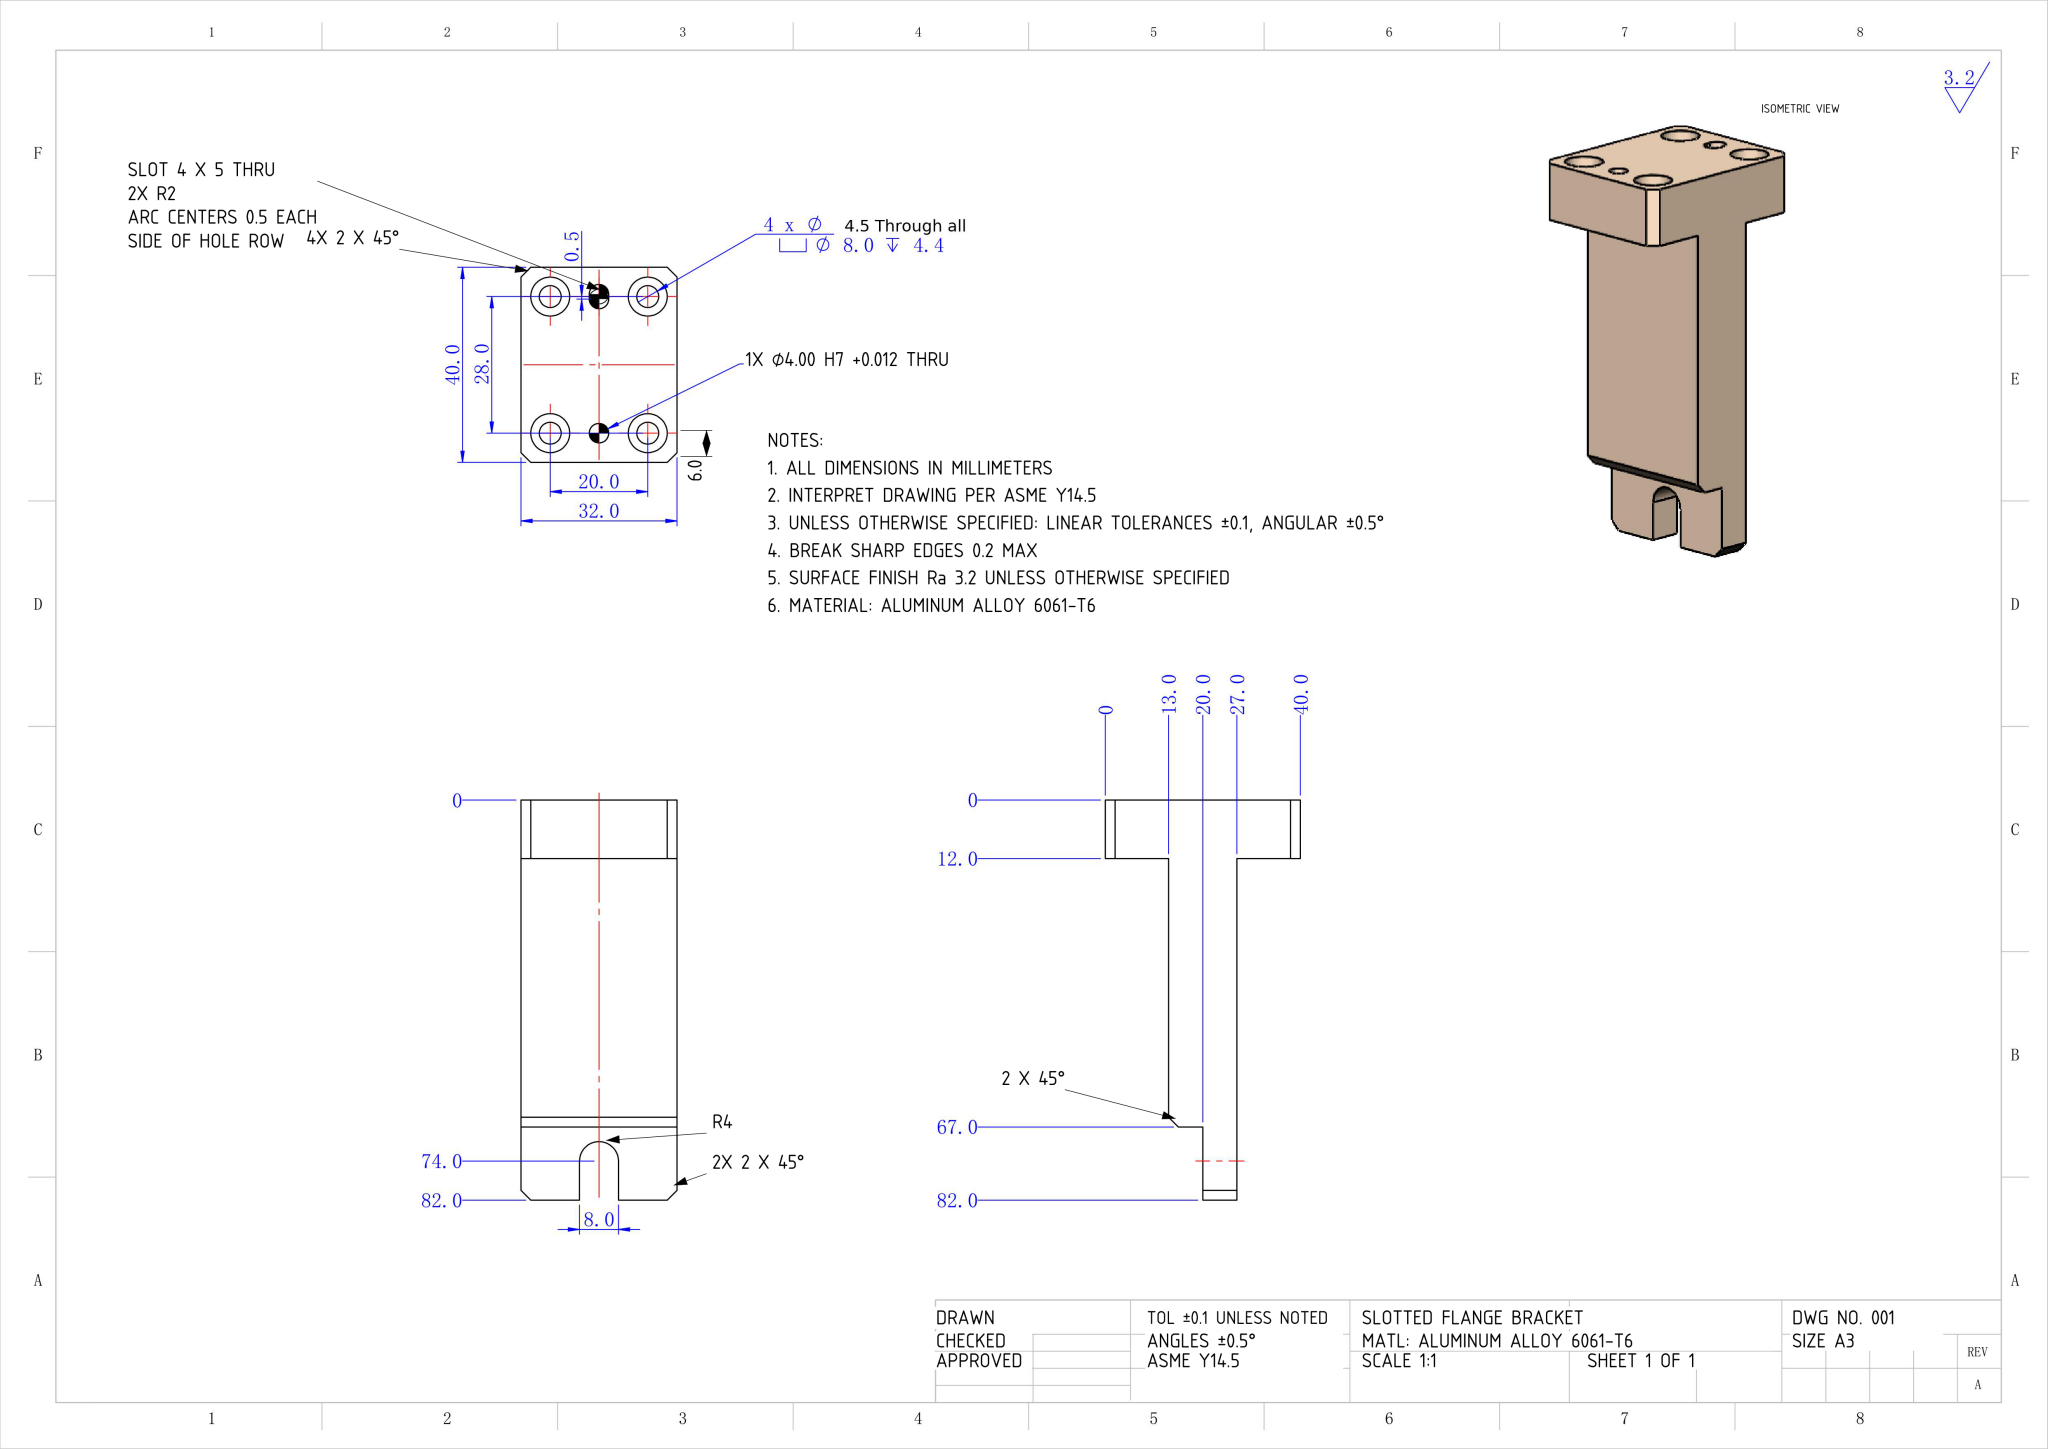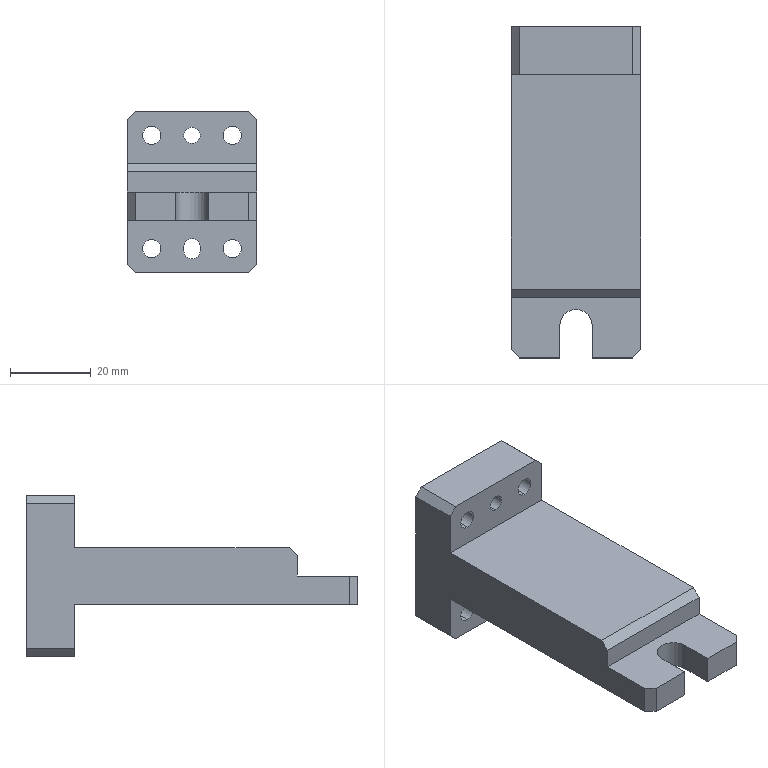Part | NX | mm | 1 solid | 50 faces | box 32 x 82 x 40 mm | volume 40830 mm3 | plane 28 | cylinder 22 | commonest cylinder face diameters 8 x9 4.5 x8 4 x5